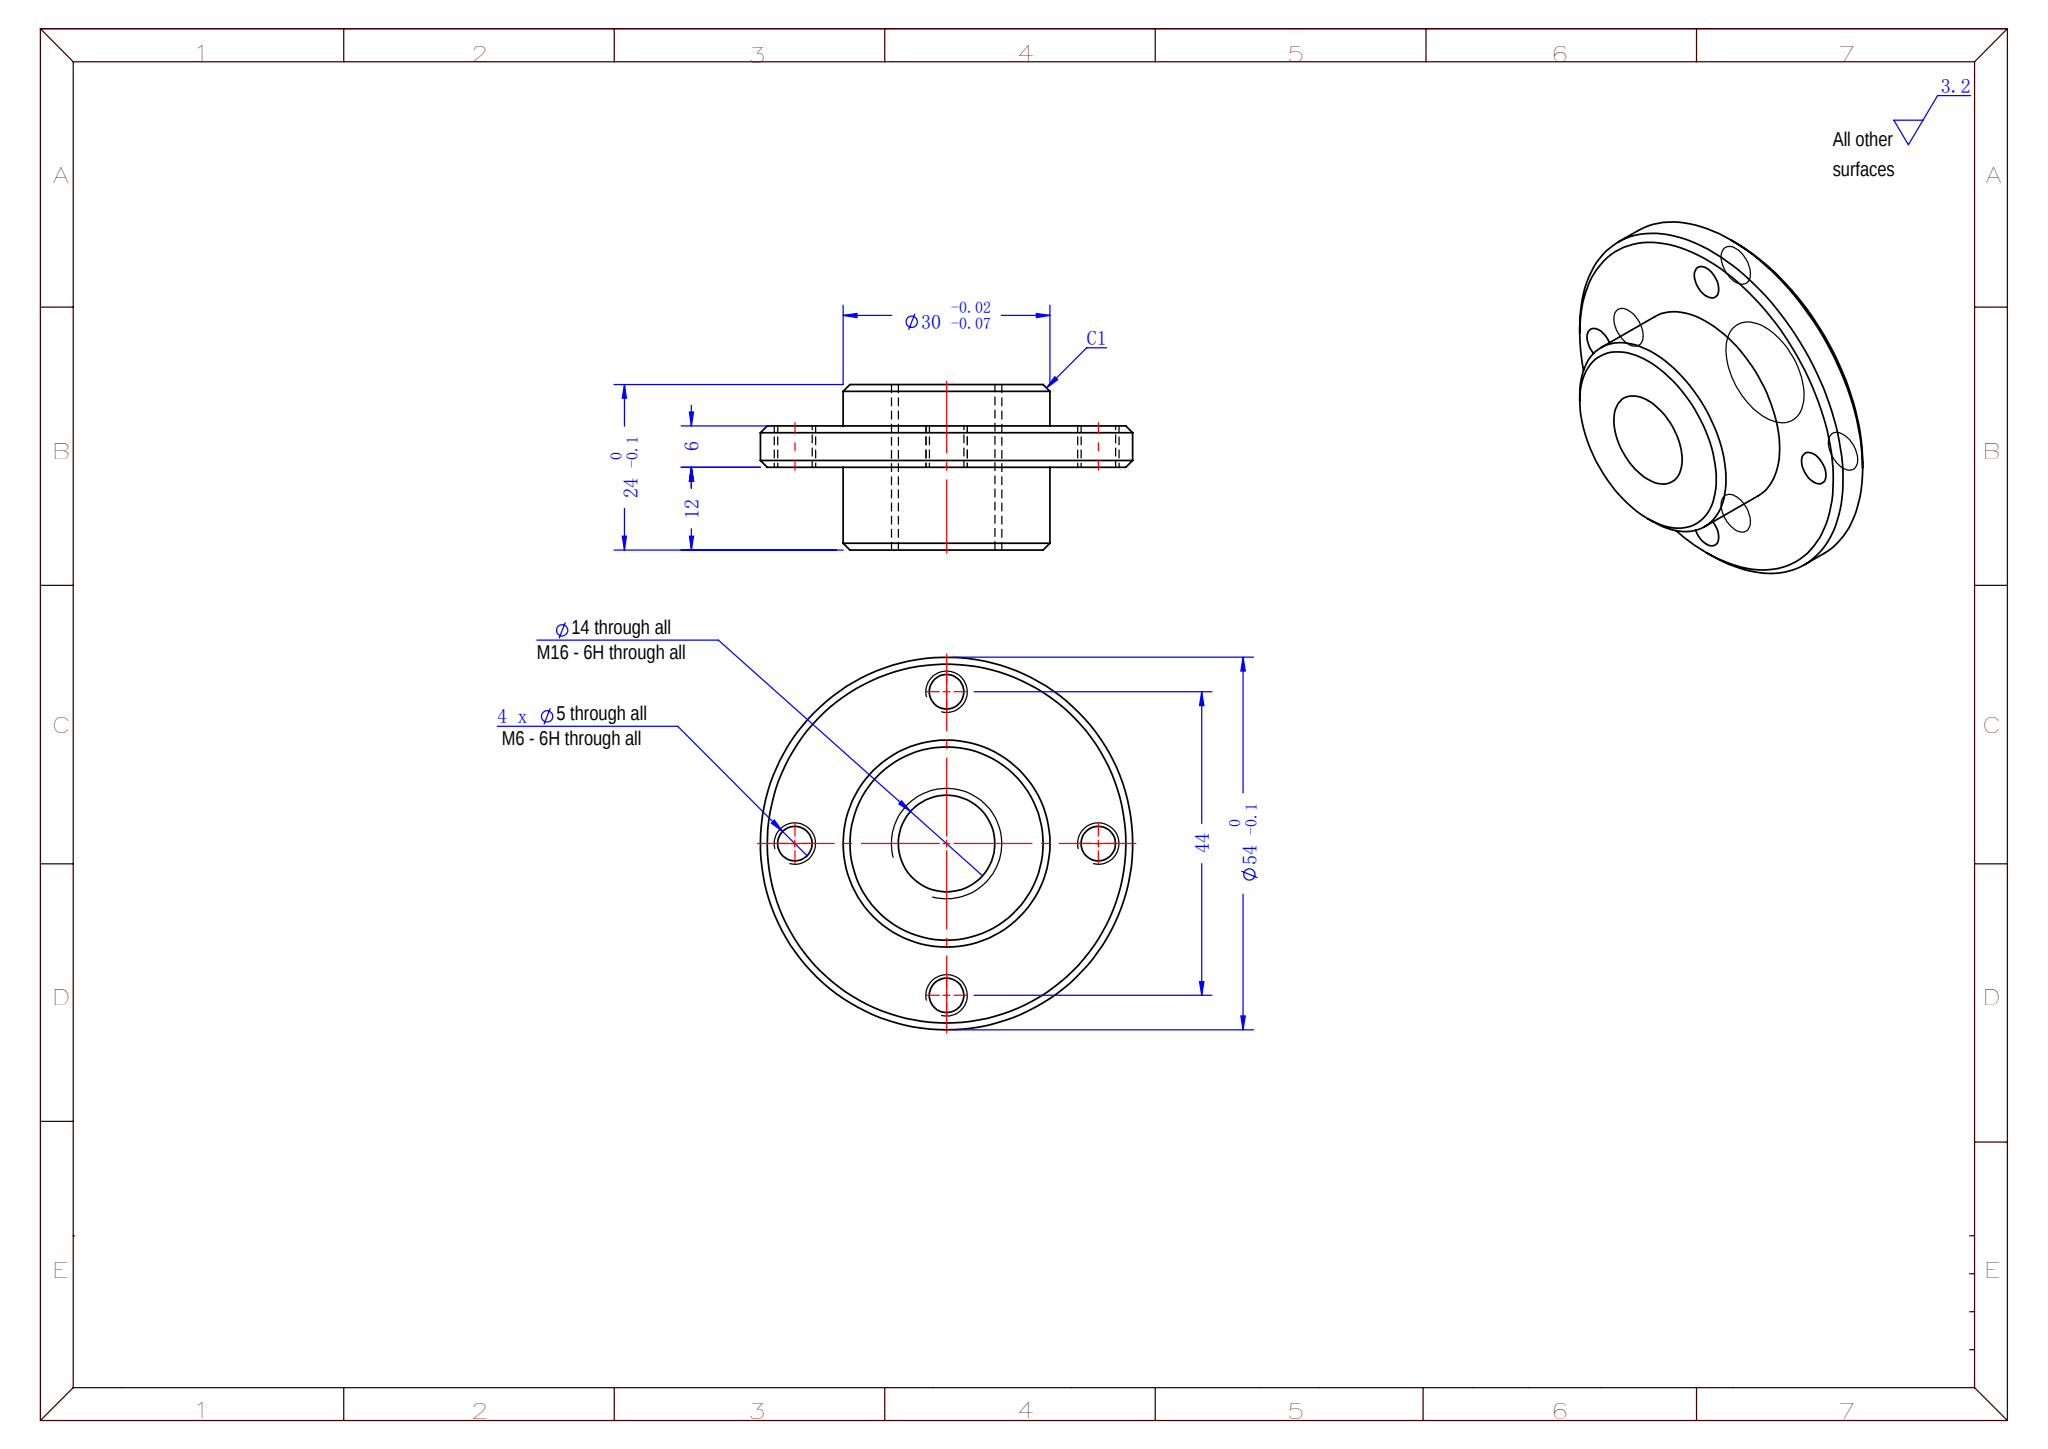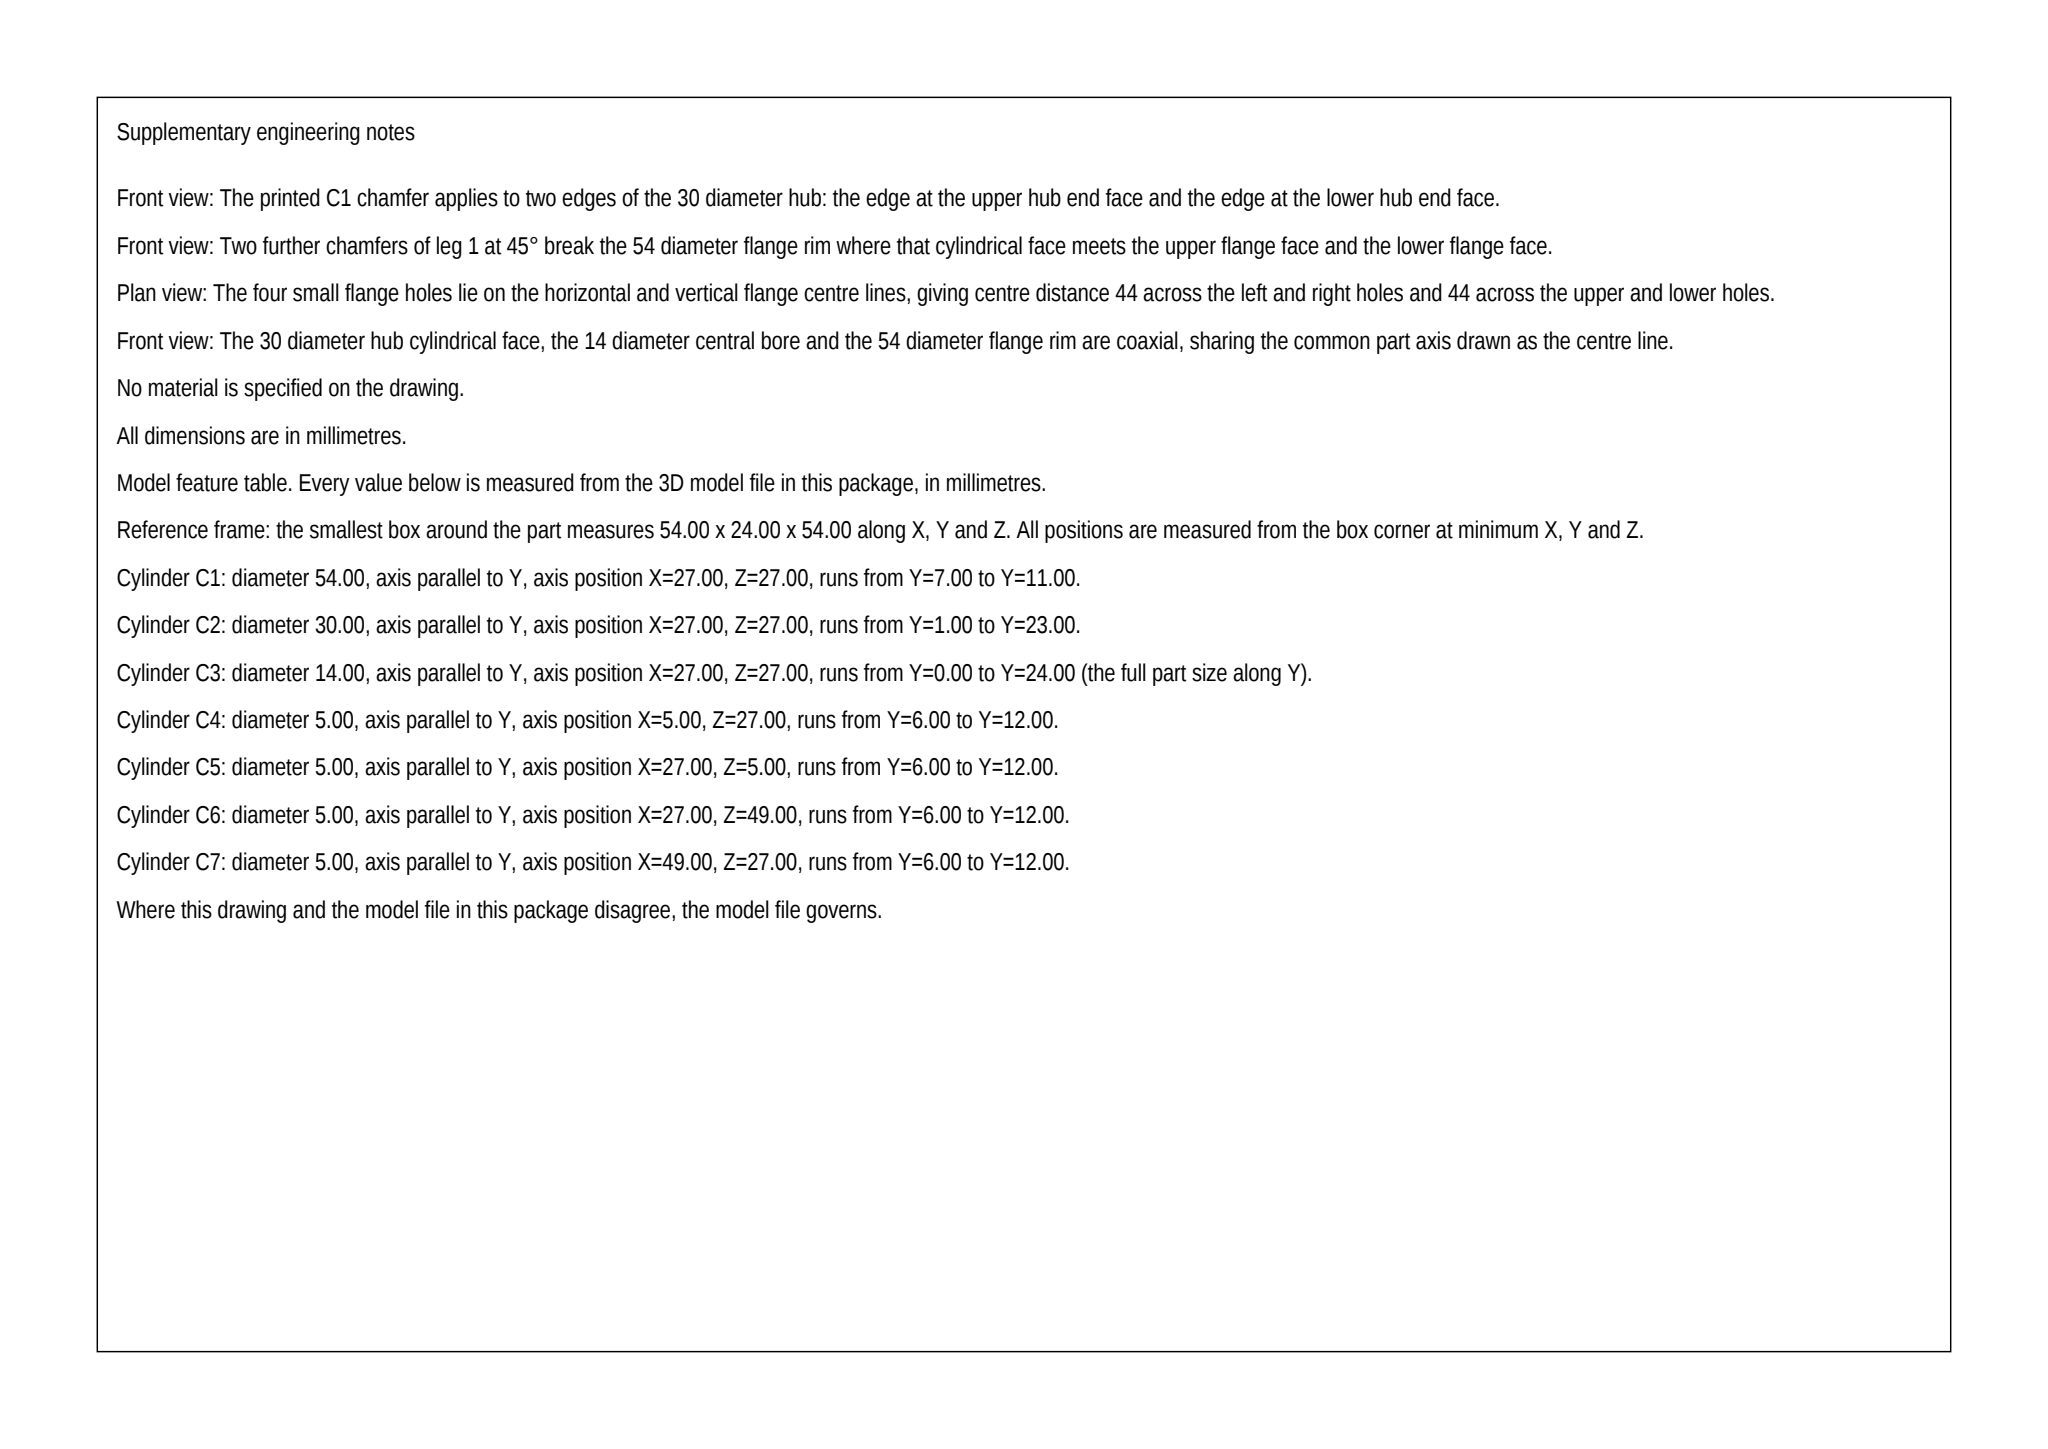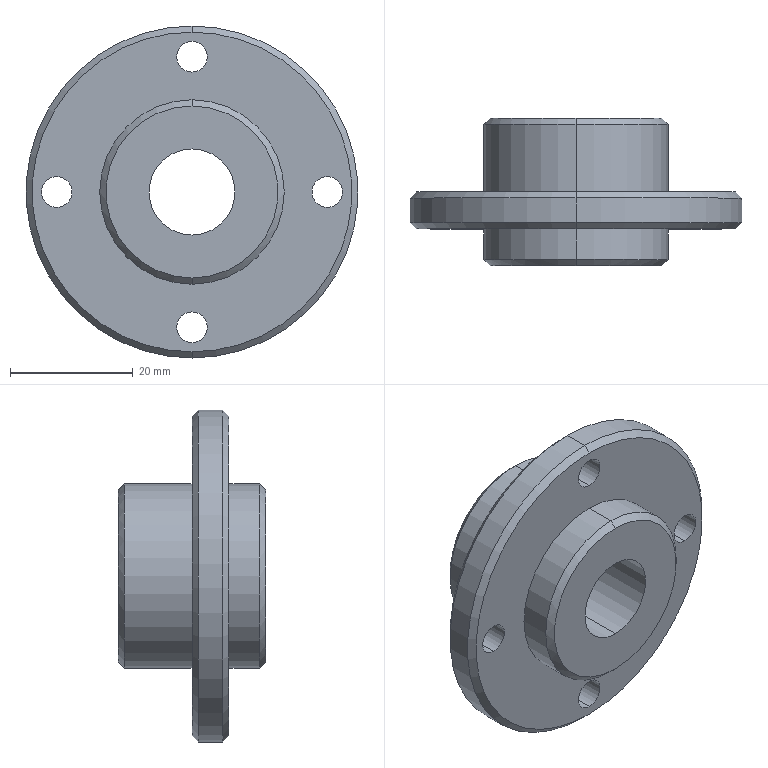Part | SolidWorks | mm | 1 solid | 28 faces | box 54 x 24 x 54 mm | volume 22039 mm3 | cylinder 16 | cone 8 | plane 4 | commonest cylinder face diameters 5 x8 30 x4 14 x2 54 x2
Drawing notes:
C1 BOTH ENDS OF Ø30 BOSS | from the solid: cones 90° incl, ref dia 28 on Ø30 cyl ends (y=0 & y=24), 4 faces
C1 BOTH OUTER EDGES OF Ø54 FLANGE (AT Y6 & Y12 FACES) | from the solid: cones 90° incl, ref dia 52 on Ø54 flange, planes y=6 and y=12
UNSPECIFIED CHAMFERS C1 | from the solid: all cones 90° incl, 1 mm leg (Ø30→28, Ø54→52); no fillets
build123d program:
from build123d import *

# Parameters (mm, degrees)
SKETCH1_R              = 27
BOSS_EXTRUDE1_DEPTH    = 12
SKETCH4_OUTSIDE_W      = 71.46
SKETCH4_OUTSIDE_H      = 71.46
SKETCH4_OUTSIDE_R      = 15
CUT_EXTRUDE3_DEPTH     = 6
SKETCH9_R              = 15
BOSS_EXTRUDE2_DEPTH    = 12
M16X1_0_TAPPED_HOLE1_D = 14
M6_TAPPED_HOLE1_D      = 5
CHAMFER1_SIZE          = 1


with BuildPart() as part:
    # Sketch1 → Boss-Extrude1 (new body)
    with BuildSketch(Plane(origin=(0, 0, 0), x_dir=(1, 0, 0), z_dir=(0, 1, 0))):
        with Locations(Location((0, 0, 0), (0, 0, 270))):
            Circle(SKETCH1_R)
    extrude(amount=BOSS_EXTRUDE1_DEPTH)

    # Sketch4 outside → Cut-Extrude3 (cut)
    with BuildSketch(Plane.XZ):
        Rectangle(SKETCH4_OUTSIDE_W, SKETCH4_OUTSIDE_H)
        with Locations(Location((0, 0, 0), (0, 0, 270))):
            Circle(SKETCH4_OUTSIDE_R, mode=Mode.SUBTRACT)
    extrude(amount=-CUT_EXTRUDE3_DEPTH, mode=Mode.SUBTRACT)

    # Sketch9 → Boss-Extrude2 (add)
    with BuildSketch(Plane(origin=(0, 12, 0), x_dir=(1, 0, 0), z_dir=(0, 1, 0))):
        with Locations(Location((0, 0, 0), (0, 0, 90))):
            Circle(SKETCH9_R)
    extrude(amount=BOSS_EXTRUDE2_DEPTH)

    # M16x1.0 Tapped Hole1 (through all)
    with Locations(Plane(origin=(0, 0, 0), x_dir=(-1, 0, 0), z_dir=(0, -1, 0))):
        with Locations((0, 0)):
            Hole(M16X1_0_TAPPED_HOLE1_D / 2)

    # M6 Tapped Hole1 (through all)
    with Locations(Plane(origin=(0, 6, 0), x_dir=(-1, 0, 0), z_dir=(0, -1, 0))):
        with Locations((-22, 0), (0, -22), (0, 22), (22, 0)):
            Hole(M6_TAPPED_HOLE1_D / 2)

    # Chamfer1
    chamfer1_edges = [part.edges().sort_by_distance(p)[0] for p in [
        (0, 0, 15),
        (0, 24, 15),
        (0, 12, -27),
        (0, 6, -27),
    ]]
    chamfer(chamfer1_edges, length=CHAMFER1_SIZE)


solid = part.part
STEP:
#1=CARTESIAN_POINT('',(0.,0.,-14.));
#2=VERTEX_POINT('',#1);
#3=CARTESIAN_POINT('',(0.,0.,14.));
#4=VERTEX_POINT('',#3);
#5=CARTESIAN_POINT('',(0.,0.,0.));
#6=DIRECTION('',(0.,-1.,0.));
#7=DIRECTION('',(0.,0.,1.));
#8=AXIS2_PLACEMENT_3D('',#5,#6,#7);
#9=CIRCLE('',#8,14.);
#10=EDGE_CURVE('',#2,#4,#9,.T.);
#11=ORIENTED_EDGE('',*,*,#10,.F.);
#12=CARTESIAN_POINT('',(0.,1.,-15.));
#13=VERTEX_POINT('',#12);
#14=CARTESIAN_POINT('',(0.,0.,-14.));
#15=DIRECTION('',(0.,0.7071,-0.7071));
#16=VECTOR('',#15,1000.);
#17=LINE('',#14,#16);
#18=EDGE_CURVE('',#2,#13,#17,.T.);
#19=ORIENTED_EDGE('',*,*,#18,.T.);
#20=CARTESIAN_POINT('',(0.,1.,15.));
#21=VERTEX_POINT('',#20);
#22=CARTESIAN_POINT('',(0.,1.,0.));
#23=DIRECTION('',(0.,1.,0.));
#24=DIRECTION('',(0.,0.,1.));
#25=AXIS2_PLACEMENT_3D('',#22,#23,#24);
#26=CIRCLE('',#25,15.);
#27=EDGE_CURVE('',#21,#13,#26,.T.);
#28=ORIENTED_EDGE('',*,*,#27,.F.);
#29=CARTESIAN_POINT('',(0.,0.,14.));
#30=DIRECTION('',(0.,0.7071,0.7071));
#31=VECTOR('',#30,1000.);
#32=LINE('',#29,#31);
#33=EDGE_CURVE('',#4,#21,#32,.T.);
#34=ORIENTED_EDGE('',*,*,#33,.F.);
#35=EDGE_LOOP('',(#11,#19,#28,#34));
#36=FACE_OUTER_BOUND('',#35,.T.);
#37=CARTESIAN_POINT('',(0.,0.,0.));
#38=DIRECTION('',(0.,1.,0.));
#39=DIRECTION('',(0.,0.,1.));
#40=AXIS2_PLACEMENT_3D('',#37,#38,#39);
#41=CONICAL_SURFACE('',#40,14.,0.7854);
#42=ADVANCED_FACE('',(#36),#41,.T.);
#43=CARTESIAN_POINT('',(0.,24.,14.));
#44=VERTEX_POINT('',#43);
#45=CARTESIAN_POINT('',(0.,24.,-14.));
#46=VERTEX_POINT('',#45);
#47=CARTESIAN_POINT('',(0.,24.,0.));
#48=DIRECTION('',(0.,1.,0.));
#49=DIRECTION('',(0.,0.,1.));
#50=AXIS2_PLACEMENT_3D('',#47,#48,#49);
#51=CIRCLE('',#50,14.);
#52=EDGE_CURVE('',#44,#46,#51,.T.);
#53=ORIENTED_EDGE('',*,*,#52,.F.);
#54=CARTESIAN_POINT('',(0.,23.,15.));
#55=VERTEX_POINT('',#54);
#56=CARTESIAN_POINT('',(0.,24.,14.));
#57=DIRECTION('',(0.,-0.7071,0.7071));
#58=VECTOR('',#57,1000.);
#59=LINE('',#56,#58);
#60=EDGE_CURVE('',#44,#55,#59,.T.);
#61=ORIENTED_EDGE('',*,*,#60,.T.);
#62=CARTESIAN_POINT('',(0.,23.,-15.));
#63=VERTEX_POINT('',#62);
#64=CARTESIAN_POINT('',(0.,23.,0.));
#65=DIRECTION('',(0.,-1.,0.));
#66=DIRECTION('',(0.,0.,1.));
#67=AXIS2_PLACEMENT_3D('',#64,#65,#66);
#68=CIRCLE('',#67,15.);
#69=EDGE_CURVE('',#63,#55,#68,.T.);
#70=ORIENTED_EDGE('',*,*,#69,.F.);
#71=CARTESIAN_POINT('',(0.,24.,-14.));
#72=DIRECTION('',(0.,-0.7071,-0.7071));
#73=VECTOR('',#72,1000.);
#74=LINE('',#71,#73);
#75=EDGE_CURVE('',#46,#63,#74,.T.);
#76=ORIENTED_EDGE('',*,*,#75,.F.);
#77=EDGE_LOOP('',(#53,#61,#70,#76));
#78=FACE_OUTER_BOUND('',#77,.T.);
#79=CARTESIAN_POINT('',(0.,24.,0.));
#80=DIRECTION('',(0.,-1.,0.));
#81=DIRECTION('',(0.,0.,-1.));
#82=AXIS2_PLACEMENT_3D('',#79,#80,#81);
#83=CONICAL_SURFACE('',#82,14.,0.7854);
#84=ADVANCED_FACE('',(#78),#83,.T.);
#85=CARTESIAN_POINT('',(0.,12.,26.));
#86=VERTEX_POINT('',#85);
#87=CARTESIAN_POINT('',(0.,12.,-26.));
#88=VERTEX_POINT('',#87);
#89=CARTESIAN_POINT('',(0.,12.,0.));
#90=DIRECTION('',(0.,1.,0.));
#91=DIRECTION('',(0.,0.,1.));
#92=AXIS2_PLACEMENT_3D('',#89,#90,#91);
#93=CIRCLE('',#92,26.);
#94=EDGE_CURVE('',#86,#88,#93,.T.);
#95=ORIENTED_EDGE('',*,*,#94,.F.);
#96=CARTESIAN_POINT('',(0.,11.,27.));
#97=VERTEX_POINT('',#96);
#98=CARTESIAN_POINT('',(0.,12.,26.));
#99=DIRECTION('',(0.,-0.7071,0.7071));
#100=VECTOR('',#99,1000.);
#101=LINE('',#98,#100);
#102=EDGE_CURVE('',#86,#97,#101,.T.);
#103=ORIENTED_EDGE('',*,*,#102,.T.);
#104=CARTESIAN_POINT('',(0.,11.,-27.));
#105=VERTEX_POINT('',#104);
#106=CARTESIAN_POINT('',(0.,11.,0.));
#107=DIRECTION('',(0.,-1.,0.));
#108=DIRECTION('',(0.,0.,1.));
#109=AXIS2_PLACEMENT_3D('',#106,#107,#108);
#110=CIRCLE('',#109,27.);
#111=EDGE_CURVE('',#105,#97,#110,.T.);
#112=ORIENTED_EDGE('',*,*,#111,.F.);
#113=CARTESIAN_POINT('',(0.,12.,-26.));
#114=DIRECTION('',(0.,-0.7071,-0.7071));
#115=VECTOR('',#114,1000.);
#116=LINE('',#113,#115);
#117=EDGE_CURVE('',#88,#105,#116,.T.);
#118=ORIENTED_EDGE('',*,*,#117,.F.);
#119=EDGE_LOOP('',(#95,#103,#112,#118));
#120=FACE_OUTER_BOUND('',#119,.T.);
#121=CARTESIAN_POINT('',(0.,12.,0.));
#122=DIRECTION('',(0.,-1.,0.));
#123=DIRECTION('',(0.,0.,-1.));
#124=AXIS2_PLACEMENT_3D('',#121,#122,#123);
#125=CONICAL_SURFACE('',#124,26.,0.7854);
#126=ADVANCED_FACE('',(#120),#125,.T.);
#127=CARTESIAN_POINT('',(0.,6.,-26.));
#128=VERTEX_POINT('',#127);
#129=CARTESIAN_POINT('',(0.,6.,26.));
#130=VERTEX_POINT('',#129);
#131=CARTESIAN_POINT('',(0.,6.,0.));
#132=DIRECTION('',(0.,-1.,0.));
#133=DIRECTION('',(0.,0.,-1.));
#134=AXIS2_PLACEMENT_3D('',#131,#132,#133);
#135=CIRCLE('',#134,26.);
#136=EDGE_CURVE('',#128,#130,#135,.T.);
#137=ORIENTED_EDGE('',*,*,#136,.F.);
#138=CARTESIAN_POINT('',(0.,7.,-27.));
#139=VERTEX_POINT('',#138);
#140=CARTESIAN_POINT('',(0.,6.,-26.));
#141=DIRECTION('',(0.,0.7071,-0.7071));
#142=VECTOR('',#141,1000.);
#143=LINE('',#140,#142);
#144=EDGE_CURVE('',#128,#139,#143,.T.);
#145=ORIENTED_EDGE('',*,*,#144,.T.);
#146=CARTESIAN_POINT('',(0.,7.,27.));
#147=VERTEX_POINT('',#146);
#148=CARTESIAN_POINT('',(0.,7.,0.));
#149=DIRECTION('',(0.,1.,0.));
#150=DIRECTION('',(0.,0.,-1.));
#151=AXIS2_PLACEMENT_3D('',#148,#149,#150);
#152=CIRCLE('',#151,27.);
#153=EDGE_CURVE('',#147,#139,#152,.T.);
#154=ORIENTED_EDGE('',*,*,#153,.F.);
#155=CARTESIAN_POINT('',(0.,6.,26.));
#156=DIRECTION('',(0.,0.7071,0.7071));
#157=VECTOR('',#156,1000.);
#158=LINE('',#155,#157);
#159=EDGE_CURVE('',#130,#147,#158,.T.);
#160=ORIENTED_EDGE('',*,*,#159,.F.);
#161=EDGE_LOOP('',(#137,#145,#154,#160));
#162=FACE_OUTER_BOUND('',#161,.T.);
#163=CARTESIAN_POINT('',(0.,6.,0.));
#164=DIRECTION('',(0.,1.,0.));
#165=DIRECTION('',(0.,0.,1.));
#166=AXIS2_PLACEMENT_3D('',#163,#164,#165);
#167=CONICAL_SURFACE('',#166,26.,0.7854);
#168=ADVANCED_FACE('',(#162),#167,.T.);
#169=CARTESIAN_POINT('',(22.,12.,-2.5));
#170=VERTEX_POINT('',#169);
#171=CARTESIAN_POINT('',(22.,12.,2.5));
#172=VERTEX_POINT('',#171);
#173=CARTESIAN_POINT('',(22.,12.,0.));
#174=DIRECTION('',(0.,1.,0.));
#175=DIRECTION('',(0.,0.,1.));
#176=AXIS2_PLACEMENT_3D('',#173,#174,#175);
#177=CIRCLE('',#176,2.5);
#178=EDGE_CURVE('',#170,#172,#177,.T.);
#179=ORIENTED_EDGE('',*,*,#178,.T.);
#180=CARTESIAN_POINT('',(22.,6.,2.5));
#181=VERTEX_POINT('',#180);
#182=CARTESIAN_POINT('',(22.,6.,2.5));
#183=DIRECTION('',(0.,-1.,0.));
#184=VECTOR('',#183,1000.);
#185=LINE('',#182,#184);
#186=EDGE_CURVE('',#172,#181,#185,.T.);
#187=ORIENTED_EDGE('',*,*,#186,.T.);
#188=CARTESIAN_POINT('',(22.,6.,-2.5));
#189=VERTEX_POINT('',#188);
#190=CARTESIAN_POINT('',(22.,6.,0.));
#191=DIRECTION('',(0.,-1.,0.));
#192=DIRECTION('',(0.,0.,-1.));
#193=AXIS2_PLACEMENT_3D('',#190,#191,#192);
#194=CIRCLE('',#193,2.5);
#195=EDGE_CURVE('',#181,#189,#194,.T.);
#196=ORIENTED_EDGE('',*,*,#195,.T.);
#197=CARTESIAN_POINT('',(22.,6.,-2.5));
#198=DIRECTION('',(0.,-1.,0.));
#199=VECTOR('',#198,1000.);
#200=LINE('',#197,#199);
#201=EDGE_CURVE('',#170,#189,#200,.T.);
#202=ORIENTED_EDGE('',*,*,#201,.F.);
#203=EDGE_LOOP('',(#179,#187,#196,#202));
#204=FACE_OUTER_BOUND('',#203,.T.);
#205=CARTESIAN_POINT('',(22.,6.,0.));
#206=DIRECTION('',(0.,-1.,0.));
#207=DIRECTION('',(0.,0.,-1.));
#208=AXIS2_PLACEMENT_3D('',#205,#206,#207);
#209=CYLINDRICAL_SURFACE('',#208,2.5);
#210=ADVANCED_FACE('',(#204),#209,.F.);
#211=CARTESIAN_POINT('',(-0.,12.,19.5));
#212=VERTEX_POINT('',#211);
#213=CARTESIAN_POINT('',(-0.,12.,24.5));
#214=VERTEX_POINT('',#213);
#215=CARTESIAN_POINT('',(-0.,12.,22.));
#216=DIRECTION('',(0.,1.,0.));
#217=DIRECTION('',(0.,0.,1.));
#218=AXIS2_PLACEMENT_3D('',#215,#216,#217);
#219=CIRCLE('',#218,2.5);
#220=EDGE_CURVE('',#212,#214,#219,.T.);
#221=ORIENTED_EDGE('',*,*,#220,.T.);
#222=CARTESIAN_POINT('',(-0.,6.,24.5));
#223=VERTEX_POINT('',#222);
#224=CARTESIAN_POINT('',(-0.,6.,24.5));
#225=DIRECTION('',(0.,-1.,0.));
#226=VECTOR('',#225,1000.);
#227=LINE('',#224,#226);
#228=EDGE_CURVE('',#214,#223,#227,.T.);
#229=ORIENTED_EDGE('',*,*,#228,.T.);
#230=CARTESIAN_POINT('',(-0.,6.,19.5));
#231=VERTEX_POINT('',#230);
#232=CARTESIAN_POINT('',(-0.,6.,22.));
#233=DIRECTION('',(0.,-1.,0.));
#234=DIRECTION('',(0.,0.,-1.));
#235=AXIS2_PLACEMENT_3D('',#232,#233,#234);
#236=CIRCLE('',#235,2.5);
#237=EDGE_CURVE('',#223,#231,#236,.T.);
#238=ORIENTED_EDGE('',*,*,#237,.T.);
#239=CARTESIAN_POINT('',(-0.,6.,19.5));
#240=DIRECTION('',(0.,-1.,0.));
#241=VECTOR('',#240,1000.);
#242=LINE('',#239,#241);
#243=EDGE_CURVE('',#212,#231,#242,.T.);
#244=ORIENTED_EDGE('',*,*,#243,.F.);
#245=EDGE_LOOP('',(#221,#229,#238,#244));
#246=FACE_OUTER_BOUND('',#245,.T.);
#247=CARTESIAN_POINT('',(-0.,6.,22.));
#248=DIRECTION('',(0.,-1.,0.));
#249=DIRECTION('',(0.,0.,-1.));
#250=AXIS2_PLACEMENT_3D('',#247,#248,#249);
#251=CYLINDRICAL_SURFACE('',#250,2.5);
#252=ADVANCED_FACE('',(#246),#251,.F.);
#253=CARTESIAN_POINT('',(-0.,12.,-24.5));
#254=VERTEX_POINT('',#253);
#255=CARTESIAN_POINT('',(-0.,12.,-19.5));
#256=VERTEX_POINT('',#255);
#257=CARTESIAN_POINT('',(-0.,12.,-22.));
#258=DIRECTION('',(0.,1.,0.));
#259=DIRECTION('',(0.,0.,1.));
#260=AXIS2_PLACEMENT_3D('',#257,#258,#259);
#261=CIRCLE('',#260,2.5);
#262=EDGE_CURVE('',#254,#256,#261,.T.);
#263=ORIENTED_EDGE('',*,*,#262,.T.);
#264=CARTESIAN_POINT('',(-0.,6.,-19.5));
#265=VERTEX_POINT('',#264);
#266=CARTESIAN_POINT('',(-0.,6.,-19.5));
#267=DIRECTION('',(0.,-1.,0.));
#268=VECTOR('',#267,1000.);
#269=LINE('',#266,#268);
#270=EDGE_CURVE('',#256,#265,#269,.T.);
#271=ORIENTED_EDGE('',*,*,#270,.T.);
#272=CARTESIAN_POINT('',(-0.,6.,-24.5));
#273=VERTEX_POINT('',#272);
#274=CARTESIAN_POINT('',(-0.,6.,-22.));
#275=DIRECTION('',(0.,-1.,0.));
#276=DIRECTION('',(0.,0.,-1.));
#277=AXIS2_PLACEMENT_3D('',#274,#275,#276);
#278=CIRCLE('',#277,2.5);
#279=EDGE_CURVE('',#265,#273,#278,.T.);
#280=ORIENTED_EDGE('',*,*,#279,.T.);
#281=CARTESIAN_POINT('',(-0.,6.,-24.5));
#282=DIRECTION('',(0.,-1.,0.));
#283=VECTOR('',#282,1000.);
#284=LINE('',#281,#283);
#285=EDGE_CURVE('',#254,#273,#284,.T.);
#286=ORIENTED_EDGE('',*,*,#285,.F.);
#287=EDGE_LOOP('',(#263,#271,#280,#286));
#288=FACE_OUTER_BOUND('',#287,.T.);
#289=CARTESIAN_POINT('',(-0.,6.,-22.));
#290=DIRECTION('',(0.,-1.,0.));
#291=DIRECTION('',(0.,0.,-1.));
#292=AXIS2_PLACEMENT_3D('',#289,#290,#291);
#293=CYLINDRICAL_SURFACE('',#292,2.5);
#294=ADVANCED_FACE('',(#288),#293,.F.);
#295=CARTESIAN_POINT('',(-22.,12.,-2.5));
#296=VERTEX_POINT('',#295);
#297=CARTESIAN_POINT('',(-22.,12.,2.5));
#298=VERTEX_POINT('',#297);
#299=CARTESIAN_POINT('',(-22.,12.,0.));
#300=DIRECTION('',(0.,1.,0.));
#301=DIRECTION('',(0.,0.,1.));
#302=AXIS2_PLACEMENT_3D('',#299,#300,#301);
#303=CIRCLE('',#302,2.5);
#304=EDGE_CURVE('',#296,#298,#303,.T.);
#305=ORIENTED_EDGE('',*,*,#304,.T.);
#306=CARTESIAN_POINT('',(-22.,6.,2.5));
#307=VERTEX_POINT('',#306);
#308=CARTESIAN_POINT('',(-22.,6.,2.5));
#309=DIRECTION('',(0.,-1.,0.));
#310=VECTOR('',#309,1000.);
#311=LINE('',#308,#310);
#312=EDGE_CURVE('',#298,#307,#311,.T.);
#313=ORIENTED_EDGE('',*,*,#312,.T.);
#314=CARTESIAN_POINT('',(-22.,6.,-2.5));
#315=VERTEX_POINT('',#314);
#316=CARTESIAN_POINT('',(-22.,6.,0.));
#317=DIRECTION('',(0.,-1.,0.));
#318=DIRECTION('',(0.,0.,-1.));
#319=AXIS2_PLACEMENT_3D('',#316,#317,#318);
#320=CIRCLE('',#319,2.5);
#321=EDGE_CURVE('',#307,#315,#320,.T.);
#322=ORIENTED_EDGE('',*,*,#321,.T.);
#323=CARTESIAN_POINT('',(-22.,6.,-2.5));
#324=DIRECTION('',(0.,-1.,0.));
#325=VECTOR('',#324,1000.);
#326=LINE('',#323,#325);
#327=EDGE_CURVE('',#296,#315,#326,.T.);
#328=ORIENTED_EDGE('',*,*,#327,.F.);
#329=EDGE_LOOP('',(#305,#313,#322,#328));
#330=FACE_OUTER_BOUND('',#329,.T.);
#331=CARTESIAN_POINT('',(-22.,6.,0.));
#332=DIRECTION('',(0.,-1.,0.));
#333=DIRECTION('',(0.,0.,-1.));
#334=AXIS2_PLACEMENT_3D('',#331,#332,#333);
#335=CYLINDRICAL_SURFACE('',#334,2.5);
#336=ADVANCED_FACE('',(#330),#335,.F.);
#337=CARTESIAN_POINT('',(0.,24.,7.));
#338=VERTEX_POINT('',#337);
#339=CARTESIAN_POINT('',(0.,24.,-7.));
#340=VERTEX_POINT('',#339);
#341=CARTESIAN_POINT('',(0.,24.,0.));
#342=DIRECTION('',(0.,-1.,0.));
#343=DIRECTION('',(0.,0.,-1.));
#344=AXIS2_PLACEMENT_3D('',#341,#342,#343);
#345=CIRCLE('',#344,7.);
#346=EDGE_CURVE('',#338,#340,#345,.T.);
#347=ORIENTED_EDGE('',*,*,#346,.F.);
#348=CARTESIAN_POINT('',(0.,-0.,7.));
#349=VERTEX_POINT('',#348);
#350=CARTESIAN_POINT('',(0.,0.,7.));
#351=DIRECTION('',(0.,-1.,0.));
#352=VECTOR('',#351,1000.);
#353=LINE('',#350,#352);
#354=EDGE_CURVE('',#338,#349,#353,.T.);
#355=ORIENTED_EDGE('',*,*,#354,.T.);
#356=CARTESIAN_POINT('',(0.,-0.,-7.));
#357=VERTEX_POINT('',#356);
#358=CARTESIAN_POINT('',(0.,-0.,0.));
#359=DIRECTION('',(0.,-1.,0.));
#360=DIRECTION('',(0.,0.,-1.));
#361=AXIS2_PLACEMENT_3D('',#358,#359,#360);
#362=CIRCLE('',#361,7.);
#363=EDGE_CURVE('',#349,#357,#362,.T.);
#364=ORIENTED_EDGE('',*,*,#363,.T.);
#365=CARTESIAN_POINT('',(0.,0.,-7.));
#366=DIRECTION('',(0.,-1.,0.));
#367=VECTOR('',#366,1000.);
#368=LINE('',#365,#367);
#369=EDGE_CURVE('',#340,#357,#368,.T.);
#370=ORIENTED_EDGE('',*,*,#369,.F.);
#371=EDGE_LOOP('',(#347,#355,#364,#370));
#372=FACE_OUTER_BOUND('',#371,.T.);
#373=CARTESIAN_POINT('',(0.,0.,0.));
#374=DIRECTION('',(0.,-1.,0.));
#375=DIRECTION('',(0.,0.,-1.));
#376=AXIS2_PLACEMENT_3D('',#373,#374,#375);
#377=CYLINDRICAL_SURFACE('',#376,7.);
#378=ADVANCED_FACE('',(#372),#377,.F.);
#379=ORIENTED_EDGE('',*,*,#69,.T.);
#380=CARTESIAN_POINT('',(0.,12.,15.));
#381=VERTEX_POINT('',#380);
#382=CARTESIAN_POINT('',(0.,24.,15.));
#383=DIRECTION('',(0.,-1.,0.));
#384=VECTOR('',#383,1000.);
#385=LINE('',#382,#384);
#386=EDGE_CURVE('',#55,#381,#385,.T.);
#387=ORIENTED_EDGE('',*,*,#386,.T.);
#388=CARTESIAN_POINT('',(0.,12.,-15.));
#389=VERTEX_POINT('',#388);
#390=CARTESIAN_POINT('',(0.,12.,0.));
#391=DIRECTION('',(0.,1.,0.));
#392=DIRECTION('',(0.,0.,1.));
#393=AXIS2_PLACEMENT_3D('',#390,#391,#392);
#394=CIRCLE('',#393,15.);
#395=EDGE_CURVE('',#381,#389,#394,.T.);
#396=ORIENTED_EDGE('',*,*,#395,.T.);
#397=CARTESIAN_POINT('',(0.,24.,-15.));
#398=DIRECTION('',(0.,-1.,0.));
#399=VECTOR('',#398,1000.);
#400=LINE('',#397,#399);
#401=EDGE_CURVE('',#63,#389,#400,.T.);
#402=ORIENTED_EDGE('',*,*,#401,.F.);
#403=EDGE_LOOP('',(#379,#387,#396,#402));
#404=FACE_OUTER_BOUND('',#403,.T.);
#405=CARTESIAN_POINT('',(0.,24.,0.));
#406=DIRECTION('',(0.,-1.,0.));
#407=DIRECTION('',(0.,0.,-1.));
#408=AXIS2_PLACEMENT_3D('',#405,#406,#407);
#409=CYLINDRICAL_SURFACE('',#408,15.);
#410=ADVANCED_FACE('',(#404),#409,.T.);
#411=CARTESIAN_POINT('',(0.,6.,-15.));
#412=VERTEX_POINT('',#411);
#413=CARTESIAN_POINT('',(0.,6.,15.));
#414=VERTEX_POINT('',#413);
#415=CARTESIAN_POINT('',(0.,6.,0.));
#416=DIRECTION('',(0.,-1.,0.));
#417=DIRECTION('',(0.,0.,-1.));
#418=AXIS2_PLACEMENT_3D('',#415,#416,#417);
#419=CIRCLE('',#418,15.);
#420=EDGE_CURVE('',#412,#414,#419,.T.);
#421=ORIENTED_EDGE('',*,*,#420,.T.);
#422=CARTESIAN_POINT('',(0.,6.,15.));
#423=DIRECTION('',(0.,-1.,0.));
#424=VECTOR('',#423,1000.);
#425=LINE('',#422,#424);
#426=EDGE_CURVE('',#414,#21,#425,.T.);
#427=ORIENTED_EDGE('',*,*,#426,.T.);
#428=ORIENTED_EDGE('',*,*,#27,.T.);
#429=CARTESIAN_POINT('',(0.,6.,-15.));
#430=DIRECTION('',(0.,-1.,0.));
#431=VECTOR('',#430,1000.);
#432=LINE('',#429,#431);
#433=EDGE_CURVE('',#412,#13,#432,.T.);
#434=ORIENTED_EDGE('',*,*,#433,.F.);
#435=EDGE_LOOP('',(#421,#427,#428,#434));
#436=FACE_OUTER_BOUND('',#435,.T.);
#437=CARTESIAN_POINT('',(0.,6.,0.));
#438=DIRECTION('',(0.,-1.,0.));
#439=DIRECTION('',(0.,0.,-1.));
#440=AXIS2_PLACEMENT_3D('',#437,#438,#439);
#441=CYLINDRICAL_SURFACE('',#440,15.);
#442=ADVANCED_FACE('',(#436),#441,.T.);
#443=ORIENTED_EDGE('',*,*,#111,.T.);
#444=CARTESIAN_POINT('',(0.,12.,27.));
#445=DIRECTION('',(0.,-1.,0.));
#446=VECTOR('',#445,1000.);
#447=LINE('',#444,#446);
#448=EDGE_CURVE('',#97,#147,#447,.T.);
#449=ORIENTED_EDGE('',*,*,#448,.T.);
#450=ORIENTED_EDGE('',*,*,#153,.T.);
#451=CARTESIAN_POINT('',(0.,12.,-27.));
#452=DIRECTION('',(0.,-1.,0.));
#453=VECTOR('',#452,1000.);
#454=LINE('',#451,#453);
#455=EDGE_CURVE('',#105,#139,#454,.T.);
#456=ORIENTED_EDGE('',*,*,#455,.F.);
#457=EDGE_LOOP('',(#443,#449,#450,#456));
#458=FACE_OUTER_BOUND('',#457,.T.);
#459=CARTESIAN_POINT('',(0.,12.,0.));
#460=DIRECTION('',(0.,-1.,0.));
#461=DIRECTION('',(0.,0.,-1.));
#462=AXIS2_PLACEMENT_3D('',#459,#460,#461);
#463=CYLINDRICAL_SURFACE('',#462,27.);
#464=ADVANCED_FACE('',(#458),#463,.T.);
#465=ORIENTED_EDGE('',*,*,#448,.F.);
#466=CARTESIAN_POINT('',(0.,11.,0.));
#467=DIRECTION('',(0.,-1.,0.));
#468=DIRECTION('',(0.,0.,1.));
#469=AXIS2_PLACEMENT_3D('',#466,#467,#468);
#470=CIRCLE('',#469,27.);
#471=EDGE_CURVE('',#97,#105,#470,.T.);
#472=ORIENTED_EDGE('',*,*,#471,.T.);
#473=ORIENTED_EDGE('',*,*,#455,.T.);
#474=CARTESIAN_POINT('',(0.,7.,0.));
#475=DIRECTION('',(0.,1.,0.));
#476=DIRECTION('',(0.,0.,-1.));
#477=AXIS2_PLACEMENT_3D('',#474,#475,#476);
#478=CIRCLE('',#477,27.);
#479=EDGE_CURVE('',#139,#147,#478,.T.);
#480=ORIENTED_EDGE('',*,*,#479,.T.);
#481=EDGE_LOOP('',(#465,#472,#473,#480));
#482=FACE_OUTER_BOUND('',#481,.T.);
#483=CARTESIAN_POINT('',(0.,12.,0.));
#484=DIRECTION('',(0.,-1.,0.));
#485=DIRECTION('',(0.,0.,-1.));
#486=AXIS2_PLACEMENT_3D('',#483,#484,#485);
#487=CYLINDRICAL_SURFACE('',#486,27.);
#488=ADVANCED_FACE('',(#482),#487,.T.);
#489=CARTESIAN_POINT('',(0.,12.,0.));
#490=DIRECTION('',(0.,1.,0.));
#491=DIRECTION('',(0.,0.,1.));
#492=AXIS2_PLACEMENT_3D('',#489,#490,#491);
#493=CIRCLE('',#492,26.);
#494=EDGE_CURVE('',#88,#86,#493,.T.);
#495=ORIENTED_EDGE('',*,*,#494,.T.);
#496=ORIENTED_EDGE('',*,*,#94,.T.);
#497=EDGE_LOOP('',(#495,#496));
#498=FACE_OUTER_BOUND('',#497,.T.);
#499=ORIENTED_EDGE('',*,*,#178,.F.);
#500=CARTESIAN_POINT('',(22.,12.,0.));
#501=DIRECTION('',(0.,1.,0.));
#502=DIRECTION('',(0.,0.,1.));
#503=AXIS2_PLACEMENT_3D('',#500,#501,#502);
#504=CIRCLE('',#503,2.5);
#505=EDGE_CURVE('',#172,#170,#504,.T.);
#506=ORIENTED_EDGE('',*,*,#505,.F.);
#507=EDGE_LOOP('',(#499,#506));
#508=FACE_BOUND('',#507,.T.);
#509=ORIENTED_EDGE('',*,*,#220,.F.);
#510=CARTESIAN_POINT('',(-0.,12.,22.));
#511=DIRECTION('',(0.,1.,0.));
#512=DIRECTION('',(0.,0.,1.));
#513=AXIS2_PLACEMENT_3D('',#510,#511,#512);
#514=CIRCLE('',#513,2.5);
#515=EDGE_CURVE('',#214,#212,#514,.T.);
#516=ORIENTED_EDGE('',*,*,#515,.F.);
#517=EDGE_LOOP('',(#509,#516));
#518=FACE_BOUND('',#517,.T.);
#519=ORIENTED_EDGE('',*,*,#262,.F.);
#520=CARTESIAN_POINT('',(-0.,12.,-22.));
#521=DIRECTION('',(0.,1.,0.));
#522=DIRECTION('',(0.,0.,1.));
#523=AXIS2_PLACEMENT_3D('',#520,#521,#522);
#524=CIRCLE('',#523,2.5);
#525=EDGE_CURVE('',#256,#254,#524,.T.);
#526=ORIENTED_EDGE('',*,*,#525,.F.);
#527=EDGE_LOOP('',(#519,#526));
#528=FACE_BOUND('',#527,.T.);
#529=ORIENTED_EDGE('',*,*,#304,.F.);
#530=CARTESIAN_POINT('',(-22.,12.,0.));
#531=DIRECTION('',(0.,1.,0.));
#532=DIRECTION('',(0.,0.,1.));
#533=AXIS2_PLACEMENT_3D('',#530,#531,#532);
#534=CIRCLE('',#533,2.5);
#535=EDGE_CURVE('',#298,#296,#534,.T.);
#536=ORIENTED_EDGE('',*,*,#535,.F.);
#537=EDGE_LOOP('',(#529,#536));
#538=FACE_BOUND('',#537,.T.);
#539=CARTESIAN_POINT('',(0.,12.,0.));
#540=DIRECTION('',(0.,1.,0.));
#541=DIRECTION('',(0.,0.,1.));
#542=AXIS2_PLACEMENT_3D('',#539,#540,#541);
#543=CIRCLE('',#542,15.);
#544=EDGE_CURVE('',#389,#381,#543,.T.);
#545=ORIENTED_EDGE('',*,*,#544,.F.);
#546=ORIENTED_EDGE('',*,*,#395,.F.);
#547=EDGE_LOOP('',(#545,#546));
#548=FACE_BOUND('',#547,.T.);
#549=CARTESIAN_POINT('',(0.,12.,0.));
#550=DIRECTION('',(0.,1.,0.));
#551=DIRECTION('',(0.,0.,1.));
#552=AXIS2_PLACEMENT_3D('',#549,#550,#551);
#553=PLANE('',#552);
#554=ADVANCED_FACE('',(#498,#508,#518,#528,#538,#548),#553,.T.);
#555=CARTESIAN_POINT('',(0.,6.,0.));
#556=DIRECTION('',(0.,-1.,0.));
#557=DIRECTION('',(0.,0.,-1.));
#558=AXIS2_PLACEMENT_3D('',#555,#556,#557);
#559=CIRCLE('',#558,26.);
#560=EDGE_CURVE('',#130,#128,#559,.T.);
#561=ORIENTED_EDGE('',*,*,#560,.T.);
#562=ORIENTED_EDGE('',*,*,#136,.T.);
#563=EDGE_LOOP('',(#561,#562));
#564=FACE_OUTER_BOUND('',#563,.T.);
#565=CARTESIAN_POINT('',(22.,6.,0.));
#566=DIRECTION('',(0.,-1.,0.));
#567=DIRECTION('',(0.,0.,-1.));
#568=AXIS2_PLACEMENT_3D('',#565,#566,#567);
#569=CIRCLE('',#568,2.5);
#570=EDGE_CURVE('',#189,#181,#569,.T.);
#571=ORIENTED_EDGE('',*,*,#570,.F.);
#572=ORIENTED_EDGE('',*,*,#195,.F.);
#573=EDGE_LOOP('',(#571,#572));
#574=FACE_BOUND('',#573,.T.);
#575=CARTESIAN_POINT('',(-0.,6.,22.));
#576=DIRECTION('',(0.,-1.,0.));
#577=DIRECTION('',(0.,0.,-1.));
#578=AXIS2_PLACEMENT_3D('',#575,#576,#577);
#579=CIRCLE('',#578,2.5);
#580=EDGE_CURVE('',#231,#223,#579,.T.);
#581=ORIENTED_EDGE('',*,*,#580,.F.);
#582=ORIENTED_EDGE('',*,*,#237,.F.);
#583=EDGE_LOOP('',(#581,#582));
#584=FACE_BOUND('',#583,.T.);
#585=CARTESIAN_POINT('',(-0.,6.,-22.));
#586=DIRECTION('',(0.,-1.,0.));
#587=DIRECTION('',(0.,0.,-1.));
#588=AXIS2_PLACEMENT_3D('',#585,#586,#587);
#589=CIRCLE('',#588,2.5);
#590=EDGE_CURVE('',#273,#265,#589,.T.);
#591=ORIENTED_EDGE('',*,*,#590,.F.);
#592=ORIENTED_EDGE('',*,*,#279,.F.);
#593=EDGE_LOOP('',(#591,#592));
#594=FACE_BOUND('',#593,.T.);
#595=CARTESIAN_POINT('',(-22.,6.,0.));
#596=DIRECTION('',(0.,-1.,0.));
#597=DIRECTION('',(0.,0.,-1.));
#598=AXIS2_PLACEMENT_3D('',#595,#596,#597);
#599=CIRCLE('',#598,2.5);
#600=EDGE_CURVE('',#315,#307,#599,.T.);
#601=ORIENTED_EDGE('',*,*,#600,.F.);
#602=ORIENTED_EDGE('',*,*,#321,.F.);
#603=EDGE_LOOP('',(#601,#602));
#604=FACE_BOUND('',#603,.T.);
#605=ORIENTED_EDGE('',*,*,#420,.F.);
#606=CARTESIAN_POINT('',(0.,6.,0.));
#607=DIRECTION('',(0.,-1.,0.));
#608=DIRECTION('',(0.,0.,-1.));
#609=AXIS2_PLACEMENT_3D('',#606,#607,#608);
#610=CIRCLE('',#609,15.);
#611=EDGE_CURVE('',#414,#412,#610,.T.);
#612=ORIENTED_EDGE('',*,*,#611,.F.);
#613=EDGE_LOOP('',(#605,#612));
#614=FACE_BOUND('',#613,.T.);
#615=CARTESIAN_POINT('',(0.,6.,0.));
#616=DIRECTION('',(0.,-1.,0.));
#617=DIRECTION('',(0.,0.,-1.));
#618=AXIS2_PLACEMENT_3D('',#615,#616,#617);
#619=PLANE('',#618);
#620=ADVANCED_FACE('',(#564,#574,#584,#594,#604,#614),#619,.T.);
#621=ORIENTED_EDGE('',*,*,#426,.F.);
#622=ORIENTED_EDGE('',*,*,#611,.T.);
#623=ORIENTED_EDGE('',*,*,#433,.T.);
#624=CARTESIAN_POINT('',(0.,1.,0.));
#625=DIRECTION('',(0.,1.,0.));
#626=DIRECTION('',(0.,0.,1.));
#627=AXIS2_PLACEMENT_3D('',#624,#625,#626);
#628=CIRCLE('',#627,15.);
#629=EDGE_CURVE('',#13,#21,#628,.T.);
#630=ORIENTED_EDGE('',*,*,#629,.T.);
#631=EDGE_LOOP('',(#621,#622,#623,#630));
#632=FACE_OUTER_BOUND('',#631,.T.);
#633=CARTESIAN_POINT('',(0.,6.,0.));
#634=DIRECTION('',(0.,-1.,0.));
#635=DIRECTION('',(0.,0.,-1.));
#636=AXIS2_PLACEMENT_3D('',#633,#634,#635);
#637=CYLINDRICAL_SURFACE('',#636,15.);
#638=ADVANCED_FACE('',(#632),#637,.T.);
#639=CARTESIAN_POINT('',(0.,0.,0.));
#640=DIRECTION('',(0.,-1.,0.));
#641=DIRECTION('',(0.,0.,1.));
#642=AXIS2_PLACEMENT_3D('',#639,#640,#641);
#643=CIRCLE('',#642,14.);
#644=EDGE_CURVE('',#4,#2,#643,.T.);
#645=ORIENTED_EDGE('',*,*,#644,.T.);
#646=ORIENTED_EDGE('',*,*,#10,.T.);
#647=EDGE_LOOP('',(#645,#646));
#648=FACE_OUTER_BOUND('',#647,.T.);
#649=CARTESIAN_POINT('',(0.,-0.,0.));
#650=DIRECTION('',(0.,-1.,0.));
#651=DIRECTION('',(0.,0.,-1.));
#652=AXIS2_PLACEMENT_3D('',#649,#650,#651);
#653=CIRCLE('',#652,7.);
#654=EDGE_CURVE('',#357,#349,#653,.T.);
#655=ORIENTED_EDGE('',*,*,#654,.F.);
#656=ORIENTED_EDGE('',*,*,#363,.F.);
#657=EDGE_LOOP('',(#655,#656));
#658=FACE_BOUND('',#657,.T.);
#659=CARTESIAN_POINT('',(0.,0.,0.));
#660=DIRECTION('',(0.,1.,0.));
#661=DIRECTION('',(0.,0.,1.));
#662=AXIS2_PLACEMENT_3D('',#659,#660,#661);
#663=PLANE('',#662);
#664=ADVANCED_FACE('',(#648,#658),#663,.F.);
#665=ORIENTED_EDGE('',*,*,#386,.F.);
#666=CARTESIAN_POINT('',(0.,23.,0.));
#667=DIRECTION('',(0.,-1.,0.));
#668=DIRECTION('',(0.,0.,1.));
#669=AXIS2_PLACEMENT_3D('',#666,#667,#668);
#670=CIRCLE('',#669,15.);
#671=EDGE_CURVE('',#55,#63,#670,.T.);
#672=ORIENTED_EDGE('',*,*,#671,.T.);
#673=ORIENTED_EDGE('',*,*,#401,.T.);
#674=ORIENTED_EDGE('',*,*,#544,.T.);
#675=EDGE_LOOP('',(#665,#672,#673,#674));
#676=FACE_OUTER_BOUND('',#675,.T.);
#677=CARTESIAN_POINT('',(0.,24.,0.));
#678=DIRECTION('',(0.,-1.,0.));
#679=DIRECTION('',(0.,0.,-1.));
#680=AXIS2_PLACEMENT_3D('',#677,#678,#679);
#681=CYLINDRICAL_SURFACE('',#680,15.);
#682=ADVANCED_FACE('',(#676),#681,.T.);
#683=CARTESIAN_POINT('',(0.,24.,0.));
#684=DIRECTION('',(0.,1.,0.));
#685=DIRECTION('',(0.,0.,1.));
#686=AXIS2_PLACEMENT_3D('',#683,#684,#685);
#687=CIRCLE('',#686,14.);
#688=EDGE_CURVE('',#46,#44,#687,.T.);
#689=ORIENTED_EDGE('',*,*,#688,.T.);
#690=ORIENTED_EDGE('',*,*,#52,.T.);
#691=EDGE_LOOP('',(#689,#690));
#692=FACE_OUTER_BOUND('',#691,.T.);
#693=CARTESIAN_POINT('',(0.,24.,0.));
#694=DIRECTION('',(0.,-1.,0.));
#695=DIRECTION('',(0.,0.,-1.));
#696=AXIS2_PLACEMENT_3D('',#693,#694,#695);
#697=CIRCLE('',#696,7.);
#698=EDGE_CURVE('',#340,#338,#697,.T.);
#699=ORIENTED_EDGE('',*,*,#698,.T.);
#700=ORIENTED_EDGE('',*,*,#346,.T.);
#701=EDGE_LOOP('',(#699,#700));
#702=FACE_BOUND('',#701,.T.);
#703=CARTESIAN_POINT('',(0.,24.,0.));
#704=DIRECTION('',(0.,1.,0.));
#705=DIRECTION('',(0.,0.,1.));
#706=AXIS2_PLACEMENT_3D('',#703,#704,#705);
#707=PLANE('',#706);
#708=ADVANCED_FACE('',(#692,#702),#707,.T.);
#709=ORIENTED_EDGE('',*,*,#354,.F.);
#710=ORIENTED_EDGE('',*,*,#698,.F.);
#711=ORIENTED_EDGE('',*,*,#369,.T.);
#712=ORIENTED_EDGE('',*,*,#654,.T.);
#713=EDGE_LOOP('',(#709,#710,#711,#712));
#714=FACE_OUTER_BOUND('',#713,.T.);
#715=CARTESIAN_POINT('',(0.,0.,0.));
#716=DIRECTION('',(0.,-1.,0.));
#717=DIRECTION('',(0.,0.,-1.));
#718=AXIS2_PLACEMENT_3D('',#715,#716,#717);
#719=CYLINDRICAL_SURFACE('',#718,7.);
#720=ADVANCED_FACE('',(#714),#719,.F.);
#721=ORIENTED_EDGE('',*,*,#312,.F.);
#722=ORIENTED_EDGE('',*,*,#535,.T.);
#723=ORIENTED_EDGE('',*,*,#327,.T.);
#724=ORIENTED_EDGE('',*,*,#600,.T.);
#725=EDGE_LOOP('',(#721,#722,#723,#724));
#726=FACE_OUTER_BOUND('',#725,.T.);
#727=CARTESIAN_POINT('',(-22.,6.,0.));
#728=DIRECTION('',(0.,-1.,0.));
#729=DIRECTION('',(0.,0.,-1.));
#730=AXIS2_PLACEMENT_3D('',#727,#728,#729);
#731=CYLINDRICAL_SURFACE('',#730,2.5);
#732=ADVANCED_FACE('',(#726),#731,.F.);
#733=ORIENTED_EDGE('',*,*,#270,.F.);
#734=ORIENTED_EDGE('',*,*,#525,.T.);
#735=ORIENTED_EDGE('',*,*,#285,.T.);
#736=ORIENTED_EDGE('',*,*,#590,.T.);
#737=EDGE_LOOP('',(#733,#734,#735,#736));
#738=FACE_OUTER_BOUND('',#737,.T.);
#739=CARTESIAN_POINT('',(-0.,6.,-22.));
#740=DIRECTION('',(0.,-1.,0.));
#741=DIRECTION('',(0.,0.,-1.));
#742=AXIS2_PLACEMENT_3D('',#739,#740,#741);
#743=CYLINDRICAL_SURFACE('',#742,2.5);
#744=ADVANCED_FACE('',(#738),#743,.F.);
#745=ORIENTED_EDGE('',*,*,#228,.F.);
#746=ORIENTED_EDGE('',*,*,#515,.T.);
#747=ORIENTED_EDGE('',*,*,#243,.T.);
#748=ORIENTED_EDGE('',*,*,#580,.T.);
#749=EDGE_LOOP('',(#745,#746,#747,#748));
#750=FACE_OUTER_BOUND('',#749,.T.);
#751=CARTESIAN_POINT('',(-0.,6.,22.));
#752=DIRECTION('',(0.,-1.,0.));
#753=DIRECTION('',(0.,0.,-1.));
#754=AXIS2_PLACEMENT_3D('',#751,#752,#753);
#755=CYLINDRICAL_SURFACE('',#754,2.5);
#756=ADVANCED_FACE('',(#750),#755,.F.);
#757=ORIENTED_EDGE('',*,*,#186,.F.);
#758=ORIENTED_EDGE('',*,*,#505,.T.);
#759=ORIENTED_EDGE('',*,*,#201,.T.);
#760=ORIENTED_EDGE('',*,*,#570,.T.);
#761=EDGE_LOOP('',(#757,#758,#759,#760));
#762=FACE_OUTER_BOUND('',#761,.T.);
#763=CARTESIAN_POINT('',(22.,6.,0.));
#764=DIRECTION('',(0.,-1.,0.));
#765=DIRECTION('',(0.,0.,-1.));
#766=AXIS2_PLACEMENT_3D('',#763,#764,#765);
#767=CYLINDRICAL_SURFACE('',#766,2.5);
#768=ADVANCED_FACE('',(#762),#767,.F.);
#769=ORIENTED_EDGE('',*,*,#144,.F.);
#770=ORIENTED_EDGE('',*,*,#560,.F.);
#771=ORIENTED_EDGE('',*,*,#159,.T.);
#772=ORIENTED_EDGE('',*,*,#479,.F.);
#773=EDGE_LOOP('',(#769,#770,#771,#772));
#774=FACE_OUTER_BOUND('',#773,.T.);
#775=CARTESIAN_POINT('',(0.,6.,0.));
#776=DIRECTION('',(0.,1.,0.));
#777=DIRECTION('',(0.,0.,1.));
#778=AXIS2_PLACEMENT_3D('',#775,#776,#777);
#779=CONICAL_SURFACE('',#778,26.,0.7854);
#780=ADVANCED_FACE('',(#774),#779,.T.);
#781=ORIENTED_EDGE('',*,*,#102,.F.);
#782=ORIENTED_EDGE('',*,*,#494,.F.);
#783=ORIENTED_EDGE('',*,*,#117,.T.);
#784=ORIENTED_EDGE('',*,*,#471,.F.);
#785=EDGE_LOOP('',(#781,#782,#783,#784));
#786=FACE_OUTER_BOUND('',#785,.T.);
#787=CARTESIAN_POINT('',(0.,12.,0.));
#788=DIRECTION('',(0.,-1.,0.));
#789=DIRECTION('',(0.,0.,-1.));
#790=AXIS2_PLACEMENT_3D('',#787,#788,#789);
#791=CONICAL_SURFACE('',#790,26.,0.7854);
#792=ADVANCED_FACE('',(#786),#791,.T.);
#793=ORIENTED_EDGE('',*,*,#60,.F.);
#794=ORIENTED_EDGE('',*,*,#688,.F.);
#795=ORIENTED_EDGE('',*,*,#75,.T.);
#796=ORIENTED_EDGE('',*,*,#671,.F.);
#797=EDGE_LOOP('',(#793,#794,#795,#796));
#798=FACE_OUTER_BOUND('',#797,.T.);
#799=CARTESIAN_POINT('',(0.,24.,0.));
#800=DIRECTION('',(0.,-1.,0.));
#801=DIRECTION('',(0.,0.,-1.));
#802=AXIS2_PLACEMENT_3D('',#799,#800,#801);
#803=CONICAL_SURFACE('',#802,14.,0.7854);
#804=ADVANCED_FACE('',(#798),#803,.T.);
#805=ORIENTED_EDGE('',*,*,#18,.F.);
#806=ORIENTED_EDGE('',*,*,#644,.F.);
#807=ORIENTED_EDGE('',*,*,#33,.T.);
#808=ORIENTED_EDGE('',*,*,#629,.F.);
#809=EDGE_LOOP('',(#805,#806,#807,#808));
#810=FACE_OUTER_BOUND('',#809,.T.);
#811=CARTESIAN_POINT('',(0.,0.,0.));
#812=DIRECTION('',(0.,1.,0.));
#813=DIRECTION('',(0.,0.,1.));
#814=AXIS2_PLACEMENT_3D('',#811,#812,#813);
#815=CONICAL_SURFACE('',#814,14.,0.7854);
#816=ADVANCED_FACE('',(#810),#815,.T.);
#817=CLOSED_SHELL('',(#42,#84,#126,#168,#210,#252,#294,#336,#378,#410,#442,#464,#488,#554,#620,#638,#664,#682,#708,#720,#732,#744,#756,#768,#780,#792,#804,#816));
#818=MANIFOLD_SOLID_BREP('',#817);
#819=CARTESIAN_POINT('',(0.,0.,0.));
#820=DIRECTION('',(0.,0.,1.));
#821=DIRECTION('',(1.,0.,0.));
#822=AXIS2_PLACEMENT_3D('',#819,#820,#821);
#823=(LENGTH_UNIT()NAMED_UNIT(*)SI_UNIT(.MILLI.,.METRE.));
#824=UNCERTAINTY_MEASURE_WITH_UNIT(LENGTH_MEASURE(0.00001),#823,'','');
#825=(NAMED_UNIT(*)PLANE_ANGLE_UNIT()SI_UNIT($,.RADIAN.));
#826=(NAMED_UNIT(*)SI_UNIT($,.STERADIAN.)SOLID_ANGLE_UNIT());
#827=(GEOMETRIC_REPRESENTATION_CONTEXT(3)GLOBAL_UNCERTAINTY_ASSIGNED_CONTEXT((#824))GLOBAL_UNIT_ASSIGNED_CONTEXT((#823,#825,#826))REPRESENTATION_CONTEXT('',''));
#828=ADVANCED_BREP_SHAPE_REPRESENTATION('',(#818,#822),#827);